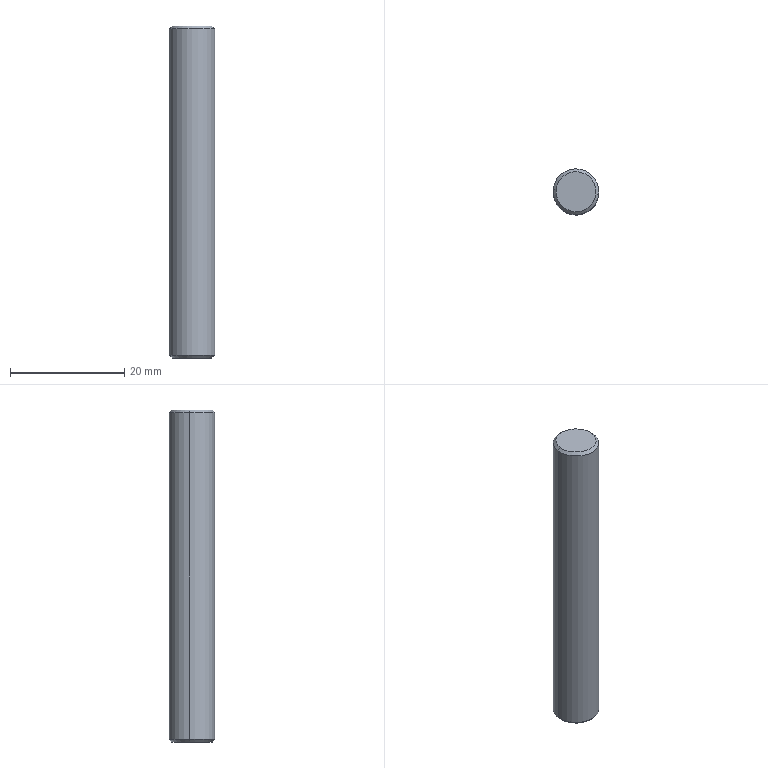Component | SolidWorks | JL001-05-03-1_JL001-05-01-008-1 | 1 solid | 8 faces | box 8 x 8 x 58 mm | volume 2909 mm3 | cone 4 | cylinder 2 | plane 2 | commonest cylinder face diameters 8 x2
build123d program:
from build123d import *

# Parameters (mm, degrees)
SKETCH1_R           = 4
BOSS_EXTRUDE1_DEPTH = 29
CHAMFER1_SIZE       = 0.5


with BuildPart() as part:
    # Sketch1 → Boss-Extrude1 (new, symmetric)
    with BuildSketch(Plane.XY):
        with Locations(Location((0, 0, 0), (0, 0, 180))):
            Circle(SKETCH1_R)
    extrude(amount=BOSS_EXTRUDE1_DEPTH, both=True)

    # Chamfer1
    chamfer1_edges = [part.edges().sort_by_distance(p)[0] for p in [
        (4, 0, -29),
        (4, 0, 29),
    ]]
    chamfer(chamfer1_edges, length=CHAMFER1_SIZE)


solid = part.part

# Placed as in the assembly
solid = solid.moved(Location((0, 294.848, 63), (0, 0, 0)))
STEP:
#1=CARTESIAN_POINT('',(0.137,11.593,3.622));
#2=VERTEX_POINT('',#1);
#3=CARTESIAN_POINT('',(-0.137,11.623,3.622));
#4=VERTEX_POINT('',#3);
#5=CARTESIAN_POINT('',(-0.,11.608,3.622));
#6=DIRECTION('',(0.,0.,1.));
#7=DIRECTION('',(0.9942,-0.1077,0.));
#8=AXIS2_PLACEMENT_3D('',#5,#6,#7);
#9=CIRCLE('',#8,0.1378);
#10=EDGE_CURVE('',#2,#4,#9,.T.);
#11=ORIENTED_EDGE('',*,*,#10,.F.);
#12=CARTESIAN_POINT('',(0.1566,11.591,3.602));
#13=VERTEX_POINT('',#12);
#14=CARTESIAN_POINT('',(0.137,11.593,3.622));
#15=DIRECTION('',(0.703,-0.07615,-0.7071));
#16=VECTOR('',#15,39.37);
#17=LINE('',#14,#16);
#18=EDGE_CURVE('',#2,#13,#17,.T.);
#19=ORIENTED_EDGE('',*,*,#18,.T.);
#20=CARTESIAN_POINT('',(-0.1566,11.625,3.602));
#21=VERTEX_POINT('',#20);
#22=CARTESIAN_POINT('',(-0.,11.608,3.602));
#23=DIRECTION('',(0.,0.,-1.));
#24=DIRECTION('',(0.9942,-0.1077,0.));
#25=AXIS2_PLACEMENT_3D('',#22,#23,#24);
#26=CIRCLE('',#25,0.1575);
#27=EDGE_CURVE('',#21,#13,#26,.T.);
#28=ORIENTED_EDGE('',*,*,#27,.F.);
#29=CARTESIAN_POINT('',(-0.137,11.623,3.622));
#30=DIRECTION('',(-0.703,0.07615,-0.7071));
#31=VECTOR('',#30,39.37);
#32=LINE('',#29,#31);
#33=EDGE_CURVE('',#4,#21,#32,.T.);
#34=ORIENTED_EDGE('',*,*,#33,.F.);
#35=EDGE_LOOP('',(#11,#19,#28,#34));
#36=FACE_OUTER_BOUND('',#35,.T.);
#37=CARTESIAN_POINT('',(-0.,11.608,3.622));
#38=DIRECTION('',(0.,0.,-1.));
#39=DIRECTION('',(-0.9942,0.1077,0.));
#40=AXIS2_PLACEMENT_3D('',#37,#38,#39);
#41=CONICAL_SURFACE('',#40,0.1378,0.7854);
#42=ADVANCED_FACE('',(#36),#41,.T.);
#43=CARTESIAN_POINT('',(-0.137,11.623,1.339));
#44=VERTEX_POINT('',#43);
#45=CARTESIAN_POINT('',(0.137,11.593,1.339));
#46=VERTEX_POINT('',#45);
#47=CARTESIAN_POINT('',(-0.,11.608,1.339));
#48=DIRECTION('',(0.,0.,-1.));
#49=DIRECTION('',(0.9942,-0.1077,0.));
#50=AXIS2_PLACEMENT_3D('',#47,#48,#49);
#51=CIRCLE('',#50,0.1378);
#52=EDGE_CURVE('',#44,#46,#51,.T.);
#53=ORIENTED_EDGE('',*,*,#52,.F.);
#54=CARTESIAN_POINT('',(-0.1566,11.625,1.358));
#55=VERTEX_POINT('',#54);
#56=CARTESIAN_POINT('',(-0.1566,11.625,1.358));
#57=DIRECTION('',(-0.703,0.07615,0.7071));
#58=VECTOR('',#57,39.37);
#59=LINE('',#56,#58);
#60=EDGE_CURVE('',#44,#55,#59,.T.);
#61=ORIENTED_EDGE('',*,*,#60,.T.);
#62=CARTESIAN_POINT('',(0.1566,11.591,1.358));
#63=VERTEX_POINT('',#62);
#64=CARTESIAN_POINT('',(-0.,11.608,1.358));
#65=DIRECTION('',(0.,0.,1.));
#66=DIRECTION('',(0.9942,-0.1077,0.));
#67=AXIS2_PLACEMENT_3D('',#64,#65,#66);
#68=CIRCLE('',#67,0.1575);
#69=EDGE_CURVE('',#63,#55,#68,.T.);
#70=ORIENTED_EDGE('',*,*,#69,.F.);
#71=CARTESIAN_POINT('',(0.1566,11.591,1.358));
#72=DIRECTION('',(0.703,-0.07615,0.7071));
#73=VECTOR('',#72,39.37);
#74=LINE('',#71,#73);
#75=EDGE_CURVE('',#46,#63,#74,.T.);
#76=ORIENTED_EDGE('',*,*,#75,.F.);
#77=EDGE_LOOP('',(#53,#61,#70,#76));
#78=FACE_OUTER_BOUND('',#77,.T.);
#79=CARTESIAN_POINT('',(-0.,11.608,1.358));
#80=DIRECTION('',(0.,0.,1.));
#81=DIRECTION('',(0.9942,-0.1077,0.));
#82=AXIS2_PLACEMENT_3D('',#79,#80,#81);
#83=CONICAL_SURFACE('',#82,0.1575,0.7854);
#84=ADVANCED_FACE('',(#78),#83,.T.);
#85=ORIENTED_EDGE('',*,*,#27,.T.);
#86=CARTESIAN_POINT('',(0.1566,11.591,3.622));
#87=DIRECTION('',(0.,0.,-1.));
#88=VECTOR('',#87,39.37);
#89=LINE('',#86,#88);
#90=EDGE_CURVE('',#13,#63,#89,.T.);
#91=ORIENTED_EDGE('',*,*,#90,.T.);
#92=ORIENTED_EDGE('',*,*,#69,.T.);
#93=CARTESIAN_POINT('',(-0.1566,11.625,3.622));
#94=DIRECTION('',(0.,0.,-1.));
#95=VECTOR('',#94,39.37);
#96=LINE('',#93,#95);
#97=EDGE_CURVE('',#21,#55,#96,.T.);
#98=ORIENTED_EDGE('',*,*,#97,.F.);
#99=EDGE_LOOP('',(#85,#91,#92,#98));
#100=FACE_OUTER_BOUND('',#99,.T.);
#101=CARTESIAN_POINT('',(-0.,11.608,3.622));
#102=DIRECTION('',(0.,0.,-1.));
#103=DIRECTION('',(-0.9942,0.1077,0.));
#104=AXIS2_PLACEMENT_3D('',#101,#102,#103);
#105=CYLINDRICAL_SURFACE('',#104,0.1575);
#106=ADVANCED_FACE('',(#100),#105,.T.);
#107=ORIENTED_EDGE('',*,*,#90,.F.);
#108=CARTESIAN_POINT('',(-0.,11.608,3.602));
#109=DIRECTION('',(0.,0.,-1.));
#110=DIRECTION('',(0.9942,-0.1077,0.));
#111=AXIS2_PLACEMENT_3D('',#108,#109,#110);
#112=CIRCLE('',#111,0.1575);
#113=EDGE_CURVE('',#13,#21,#112,.T.);
#114=ORIENTED_EDGE('',*,*,#113,.T.);
#115=ORIENTED_EDGE('',*,*,#97,.T.);
#116=CARTESIAN_POINT('',(-0.,11.608,1.358));
#117=DIRECTION('',(0.,0.,1.));
#118=DIRECTION('',(0.9942,-0.1077,0.));
#119=AXIS2_PLACEMENT_3D('',#116,#117,#118);
#120=CIRCLE('',#119,0.1575);
#121=EDGE_CURVE('',#55,#63,#120,.T.);
#122=ORIENTED_EDGE('',*,*,#121,.T.);
#123=EDGE_LOOP('',(#107,#114,#115,#122));
#124=FACE_OUTER_BOUND('',#123,.T.);
#125=CARTESIAN_POINT('',(-0.,11.608,3.622));
#126=DIRECTION('',(0.,0.,-1.));
#127=DIRECTION('',(-0.9942,0.1077,0.));
#128=AXIS2_PLACEMENT_3D('',#125,#126,#127);
#129=CYLINDRICAL_SURFACE('',#128,0.1575);
#130=ADVANCED_FACE('',(#124),#129,.T.);
#131=CARTESIAN_POINT('',(-0.,11.608,3.622));
#132=DIRECTION('',(0.,0.,1.));
#133=DIRECTION('',(0.9942,-0.1077,0.));
#134=AXIS2_PLACEMENT_3D('',#131,#132,#133);
#135=CIRCLE('',#134,0.1378);
#136=EDGE_CURVE('',#4,#2,#135,.T.);
#137=ORIENTED_EDGE('',*,*,#136,.T.);
#138=ORIENTED_EDGE('',*,*,#10,.T.);
#139=EDGE_LOOP('',(#137,#138));
#140=FACE_OUTER_BOUND('',#139,.T.);
#141=CARTESIAN_POINT('',(-0.,11.608,3.622));
#142=DIRECTION('',(0.,0.,1.));
#143=DIRECTION('',(0.9942,-0.1077,0.));
#144=AXIS2_PLACEMENT_3D('',#141,#142,#143);
#145=PLANE('',#144);
#146=ADVANCED_FACE('',(#140),#145,.T.);
#147=CARTESIAN_POINT('',(-0.,11.608,1.339));
#148=DIRECTION('',(0.,0.,-1.));
#149=DIRECTION('',(0.9942,-0.1077,0.));
#150=AXIS2_PLACEMENT_3D('',#147,#148,#149);
#151=CIRCLE('',#150,0.1378);
#152=EDGE_CURVE('',#46,#44,#151,.T.);
#153=ORIENTED_EDGE('',*,*,#152,.T.);
#154=ORIENTED_EDGE('',*,*,#52,.T.);
#155=EDGE_LOOP('',(#153,#154));
#156=FACE_OUTER_BOUND('',#155,.T.);
#157=CARTESIAN_POINT('',(-0.,11.608,1.339));
#158=DIRECTION('',(0.,0.,1.));
#159=DIRECTION('',(0.9942,-0.1077,0.));
#160=AXIS2_PLACEMENT_3D('',#157,#158,#159);
#161=PLANE('',#160);
#162=ADVANCED_FACE('',(#156),#161,.F.);
#163=ORIENTED_EDGE('',*,*,#60,.F.);
#164=ORIENTED_EDGE('',*,*,#152,.F.);
#165=ORIENTED_EDGE('',*,*,#75,.T.);
#166=ORIENTED_EDGE('',*,*,#121,.F.);
#167=EDGE_LOOP('',(#163,#164,#165,#166));
#168=FACE_OUTER_BOUND('',#167,.T.);
#169=CARTESIAN_POINT('',(-0.,11.608,1.358));
#170=DIRECTION('',(0.,0.,1.));
#171=DIRECTION('',(0.9942,-0.1077,0.));
#172=AXIS2_PLACEMENT_3D('',#169,#170,#171);
#173=CONICAL_SURFACE('',#172,0.1575,0.7854);
#174=ADVANCED_FACE('',(#168),#173,.T.);
#175=ORIENTED_EDGE('',*,*,#18,.F.);
#176=ORIENTED_EDGE('',*,*,#136,.F.);
#177=ORIENTED_EDGE('',*,*,#33,.T.);
#178=ORIENTED_EDGE('',*,*,#113,.F.);
#179=EDGE_LOOP('',(#175,#176,#177,#178));
#180=FACE_OUTER_BOUND('',#179,.T.);
#181=CARTESIAN_POINT('',(-0.,11.608,3.622));
#182=DIRECTION('',(0.,0.,-1.));
#183=DIRECTION('',(-0.9942,0.1077,0.));
#184=AXIS2_PLACEMENT_3D('',#181,#182,#183);
#185=CONICAL_SURFACE('',#184,0.1378,0.7854);
#186=ADVANCED_FACE('',(#180),#185,.T.);
#187=CLOSED_SHELL('',(#42,#84,#106,#130,#146,#162,#174,#186));
#188=MANIFOLD_SOLID_BREP('',#187);
#189=CARTESIAN_POINT('',(0.,0.,0.));
#190=DIRECTION('',(0.,0.,1.));
#191=DIRECTION('',(1.,0.,0.));
#192=AXIS2_PLACEMENT_3D('',#189,#190,#191);
#193=(LENGTH_UNIT()NAMED_UNIT(*)SI_UNIT($,.METRE.));
#194=LENGTH_MEASURE_WITH_UNIT(LENGTH_MEASURE(0.0254),#193);
#195=DIMENSIONAL_EXPONENTS(1.,0.,0.,0.,0.,0.,0.);
#196=(CONVERSION_BASED_UNIT('',#194)LENGTH_UNIT()NAMED_UNIT(#195));
#197=UNCERTAINTY_MEASURE_WITH_UNIT(LENGTH_MEASURE(0.00001),#196,'','');
#198=(NAMED_UNIT(*)PLANE_ANGLE_UNIT()SI_UNIT($,.RADIAN.));
#199=(NAMED_UNIT(*)SI_UNIT($,.STERADIAN.)SOLID_ANGLE_UNIT());
#200=(GEOMETRIC_REPRESENTATION_CONTEXT(3)GLOBAL_UNCERTAINTY_ASSIGNED_CONTEXT((#197))GLOBAL_UNIT_ASSIGNED_CONTEXT((#196,#198,#199))REPRESENTATION_CONTEXT('',''));
#201=ADVANCED_BREP_SHAPE_REPRESENTATION('',(#188,#192),#200);
#202=COLOUR_RGB('',0.7922,0.8196,0.9333);
#203=FILL_AREA_STYLE_COLOUR('',#202);
#204=FILL_AREA_STYLE('',(#203));
#205=SURFACE_STYLE_FILL_AREA(#204);
#206=SURFACE_SIDE_STYLE('',(#205));
#207=SURFACE_STYLE_USAGE(.BOTH.,#206);
#208=PRESENTATION_STYLE_ASSIGNMENT((#207));
#209=STYLED_ITEM('',(#208),#188);
#210=PRESENTATION_LAYER_ASSIGNMENT('','',(#209));
#211=(LENGTH_UNIT()NAMED_UNIT(*)SI_UNIT($,.METRE.));
#212=LENGTH_MEASURE_WITH_UNIT(LENGTH_MEASURE(0.0254),#211);
#213=DIMENSIONAL_EXPONENTS(1.,0.,0.,0.,0.,0.,0.);
#214=(CONVERSION_BASED_UNIT('',#212)LENGTH_UNIT()NAMED_UNIT(#213));
#215=UNCERTAINTY_MEASURE_WITH_UNIT(LENGTH_MEASURE(0.00001),#214,'','');
#216=(NAMED_UNIT(*)PLANE_ANGLE_UNIT()SI_UNIT($,.RADIAN.));
#217=(NAMED_UNIT(*)SI_UNIT($,.STERADIAN.)SOLID_ANGLE_UNIT());
#218=(GEOMETRIC_REPRESENTATION_CONTEXT(3)GLOBAL_UNCERTAINTY_ASSIGNED_CONTEXT((#215))GLOBAL_UNIT_ASSIGNED_CONTEXT((#214,#216,#217))REPRESENTATION_CONTEXT('',''));
#219=MECHANICAL_DESIGN_GEOMETRIC_PRESENTATION_REPRESENTATION('',(#209),#218);